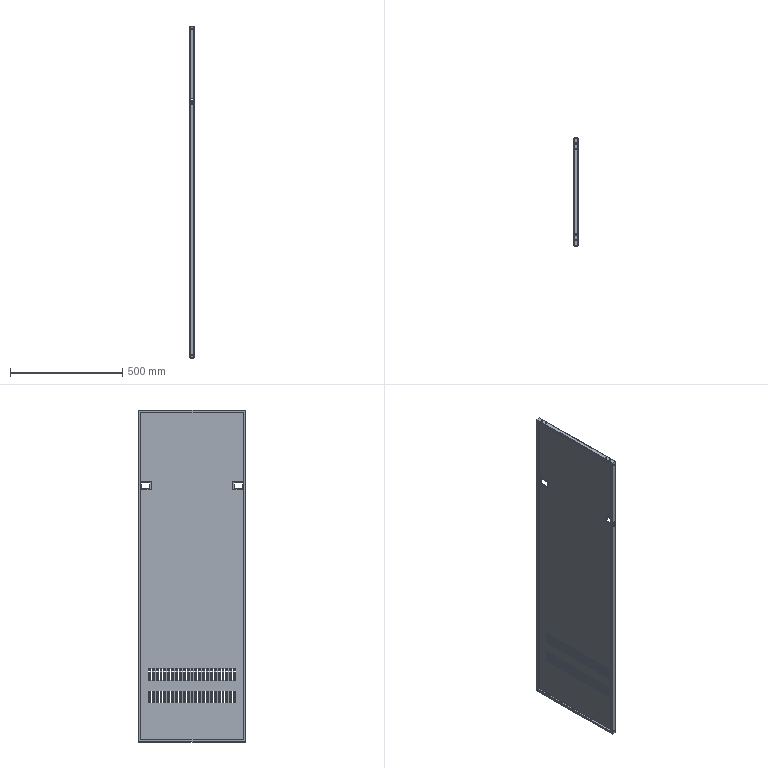Component | SolidWorks | SideDoorAssembly-2_SideDoor-1 | 1 solid | 394 faces | volume 946539 mm3 | plane 338 | cylinder 40 | spline 16 | commonest cylinder face diameters 6.5 x24 0.2 x8 2.6 x8